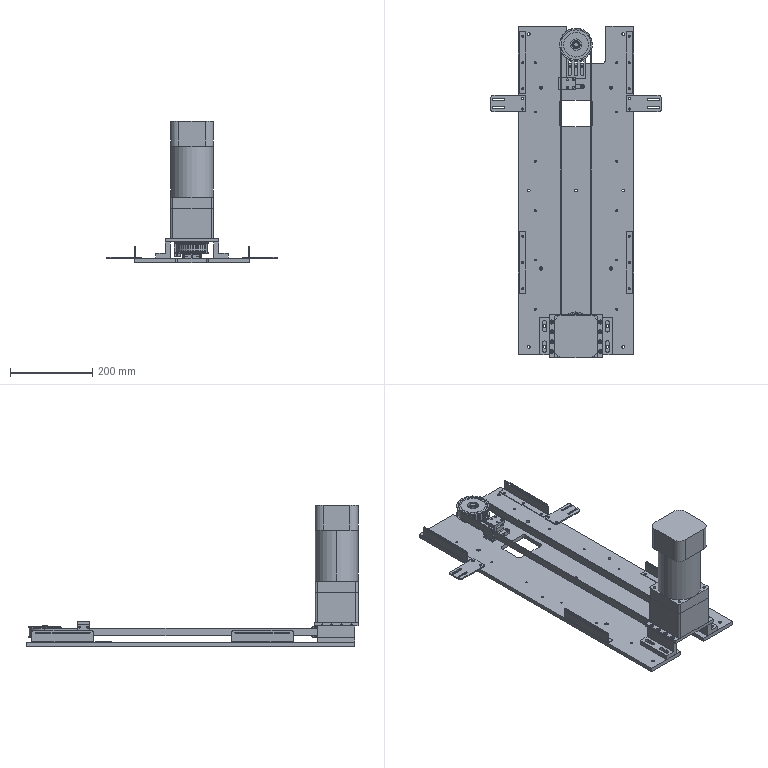Assembly | SolidWorks | mm | 20 component files | 21 solids | 990 faces | box 414 x 807.5 x 343 mm | volume 5377304 mm3 | cylinder 626 | plane 299 | cone 65 | commonest cylinder face diameters 2.94 x86 2.08 x84 5 x54 4.2 x50 10 x46 66.21 x40 71.39 x38 3.3 x36
Bill of materials:
200WBrakeMotor, | 1 |  | Vertical stacked body: square block base, a cylindrical middle section, and a square cap with rounded corners on top; a small round shaft with a short collar sticks out of the base end. The overall form looks like a motor or gearmotor housing.
ATPA18H075 | 1 |  | Toothed pulley-like wheel with flanges at both ends. The toothed cylindrical hub has many axial grooves, there is a central through bore with a counterbore or step on one face, and one radial hole goes through the toothed rim.
'-2 | 1 |  | Toothed pulley-like wheel with end flanges, similar in form to unnamed part, but with a plain bore that has a single rectangular keyway, and with radial holes through the toothed rim.
3 | 1 |  | Short solid cylinder with chamfered ends. One end has a hexagonal socket recess and the other end has a flat circular face inside a chamfer. The form looks like a set screw / grub screw.
DC-024-05 | 2 |  | L-section block: a long, tall upright wall joined to a lower base flange running its full length. The top of the wall has a row of four small holes, and the base flange has two elongated slots.
DC-024-06 | 1 |  | Flat rectangular plate with one large round through hole set toward one end. Four larger holes sit near the corners and eight smaller holes run along the two long edges.
DC-024-24 | 1 |  | Rectangular block with three parallel slots at one end and a round bore at the other. A narrow saw cut runs from the bore to the end face, and a cross hole runs through the side, which looks like a split-clamp feature. There is a step on the underside.
DC-024-25 | 1 |  | Stepped cylindrical pin: a larger-diameter base section and a longer, smaller-diameter shank. A narrow circumferential groove sits near the free end of the shank, and the edges are chamfered.
DC-024-29 | 1 |  | Thick L-shaped angle bracket. The horizontal flange has four larger through holes in a rectangular pattern, and the vertical leg has four smaller through holes in a rectangular pattern.
DC-024-30 | 1 |  | Flat rectangular plate with four round through holes, one near each corner.
DC-024-31 | 4 |  | Long, thin angle bracket (L-section). The tall vertical leg has a long slot with rounded ends running nearly its full length and rounded top corners. The short horizontal flange has three round holes along its length.
DC-024-39 | 1 |  | Rectangular bar with chamfered vertical corners, which gives an elongated octagonal outline in plan. Two vertical through holes near the ends appear counterbored, and one horizontal cross hole goes through the long side at the middle.
DC-024-40 | 1 |  | Long, thin, flat rectangular plate. Each short end has a rectangular notch with rounded corners, so the plate's outline looks roughly like an H or a double U. There is one rounded-rectangle through-cutout near one end, and many small round through-holes are spread over the face.
DC-024-43 | 2 |  | Flat rectangular plate with rounded corners. Two round through-holes sit near one short edge, and two parallel elongated slots with rounded ends run lengthwise near the opposite short edge.
tongbudai | 1 |  | Closed, thin-walled band shaped like an obround (stadium): two straight parallel sides joined by semicircular ends. It is open at the top and bottom, with no floor or cover.
Mates:
1. coincident | DC-024-05-1 face at (-90.633, -439.091, 53) dir (0, 0, 1) | DC-024-06-1 face at (-25.633, -394.091, 53) dir (0, 0, -1)
2. coincident | DC-024-05-1 face at (-90.633, -439.091, 25) dir (-1, 0, 0) | DC-024-06-1 face at (-90.633, -446.591, 61) dir (-1, 0, 0)
3. width | 200WBrakeMotor,-1 face at (26.367, -342.591, 134) dir (1, 0, 0) | 200WBrakeMotor,-1 face at (-77.633, -342.591, 134) dir (-1, 0, 0) | DC-024-05-1 face at (-90.633, -439.091, 25) dir (-1, 0, 0) | DC-024-05-2 face at (39.367, -349.091, 25) dir (1, 0, 0)
4. coincident | DC-024-06-1 face at (39.367, -446.591, 61) dir (0, -1, 0) | 200WBrakeMotor,-1 face at (-77.633, -446.591, 134) dir (0, -1, 0)
5. coincident | DC-024-06-1 face at (-25.633, -394.091, 61) dir (0, 0, 1) | 200WBrakeMotor,-1 face at (-25.633, -394.591, 61) dir (0, 0, -1)
6. coincident | ATPA18H075-A-N20-1/-2-1 face at (-22.284, -394.309, 51.5) dir (0, 0, 1) | ATPA18H075-1 face at (-43.362, 325.7, 51.5) dir (0, 0, 1)
7. concentric | DC-024-24-1 face at (-25.633, 315.409, -17.713) dir (0, 0, 1) r 7.5 | ATPA18H075-1 face at (-25.633, 315.409, 5.216) dir (0, 0, 1) r 10
8. concentric | DC-024-24-1 face at (-25.633, 315.409, -17.713) dir (0, 0, 1) r 7.5 | DC-024-25-1 face at (-25.633, 315.409, 54.5) dir (0, 0, -1) r 6
9. coincident | tongbudai-1 face at (-61.333, 315.409, 48) dir (1, 0, 0) | DC-024-29-1 face at (-61.333, 205.806, 63) dir (-1, 0, 0)
10. coincident | DC-024-29-1 face at (-61.333, 235.806, 63) dir (0, 1, 0) | DC-024-30-1 face at (-63.333, 235.806, 18) dir (0, 1, 0)
11. coincident | tongbudai-1 face at (-63.333, 315.409, 48) dir (-1, 0, 0) | DC-024-30-1 face at (-63.333, 220.806, 37) dir (1, 0, 0)
12. coincident | DC-024-29-1 face at (-53.333, 205.806, 18) dir (0, 0, -1) | DC-024-30-1 face at (-63.333, 205.806, 18) dir (0, 0, -1)
13. coincident | DC-024-31-1 face at (114.367, 196.909, 42.5) dir (1, 0, 0) | DC-024-31-2 face at (114.367, -289.091, 42.5) dir (1, 0, 0)
14. coincident | DC-024-31-1 face at (112.867, 196.909, 13) dir (0, 0, -1) | DC-024-31-2 face at (112.867, -289.091, 13) dir (0, 0, -1)
15. coincident | DC-024-05-2 face at (39.367, -349.091, 25) dir (1, 0, 0) | DC-024-06-1 face at (39.367, -446.591, 61) dir (1, 0, 0)
16. width | DC-024-05-2 face at (27.367, -439.091, 13) dir (0, -1, 0) | DC-024-05-2 face at (27.367, -349.091, 13) dir (0, 1, 0) | DC-024-06-1 face at (39.367, -341.591, 61) dir (0, 1, 0) | DC-024-06-1 face at (39.367, -446.591, 61) dir (0, -1, 0)
17. coincident | DC-024-05-2 face at (39.367, -349.091, 53) dir (0, 0, 1) | DC-024-06-1 face at (-25.633, -394.091, 53) dir (0, 0, -1)
18. coincident | DC-024-05-1 face at (-113.633, -439.091, 13) dir (0, 0, -1) | DC-024-40-1 face at (-25.633, -9.091, 13) dir (0, 0, 1)
19. coincident | DC-024-05-1 face at (-78.633, -439.091, 13) dir (0, -1, 0) | DC-024-40-1 face at (114.367, -439.091, 13) dir (0, -1, 0)
20. width | DC-024-05-2 face at (39.367, -349.091, 25) dir (1, 0, 0) | DC-024-05-1 face at (-90.633, -439.091, 25) dir (-1, 0, 0) | DC-024-40-1 face at (-165.633, -439.091, 13) dir (-1, 0, 0) | DC-024-40-1 face at (114.367, -439.091, 13) dir (1, 0, 0)
21. coincident | DC-024-31-1 face at (112.867, 196.909, 13) dir (0, 0, -1) | DC-024-40-1 face at (-25.633, -9.091, 13) dir (0, 0, 1)
22. coincident | DC-024-31-1 face at (114.367, 196.909, 42.5) dir (1, 0, 0) | DC-024-40-1 face at (114.367, -439.091, 13) dir (1, 0, 0)
23. width | DC-024-24-1 face at (-3.133, 233.409, 23.5) dir (1, 0, 0) | DC-024-24-1 face at (-48.133, 233.409, 23.5) dir (-1, 0, 0) | DC-024-40-1 face at (-165.633, -439.091, 13) dir (-1, 0, 0) | DC-024-40-1 face at (114.367, -439.091, 13) dir (1, 0, 0)
24. coincident | DC-024-24-1 face at (-25.633, 283.409, 3.5) dir (0, 0, -1) | DC-024-25-1 face at (-25.633, 315.409, 3.5) dir (0, 0, -1)
25. concentric | tongbudai-1 face at (-25.633, 315.409, 48) dir (0, 0, -1) r 37.7 | ATPA18H075-1 face at (-25.633, 315.409, 38.5) dir (0, 0, 1) r 35.695
26. width | tongbudai-1 face at (-25.633, 315.409, 48) dir (0, 0, 1) | tongbudai-1 face at (-25.633, 315.409, 29) dir (0, 0, -1) | ATPA18H075-1 face at (-56.802, 333.502, 49) dir (0, 0, -1) | ATPA18H075-1 face at (-56.802, 333.502, 28) dir (0, 0, 1)
27. concentric | ATPA18H075-A-N20-1/-2-1 face at (-25.633, -374.591, 38.5) dir (0, 0, -1) r 35.695 | tongbudai-1 face at (-25.633, -374.591, 48) dir (0, 0, -1) r 37.7
28. coincident | DC-024-40-1 face at (-25.633, -9.091, 13) dir (0, 0, 1) | DC-024-39-1 face at (-25.633, 213.409, 13) dir (0, 0, -1)
29. width | DC-024-39-1 face at (-45.633, 208.409, 23) dir (-1, 0, 0) | DC-024-39-1 face at (-5.633, 208.409, 23) dir (1, 0, 0) | DC-024-24-1 face at (-3.133, 233.409, 23.5) dir (1, 0, 0) | DC-024-24-1 face at (-48.133, 233.409, 23.5) dir (-1, 0, 0)
30. distance | DC-024-39-1 face at (-5.633, 218.409, 23) dir (0, 1, 0) | DC-024-24-1 face at (-3.133, 233.409, 23.5) dir (0, -1, 0)
31. coincident | DC-024-05-1 face at (-78.633, -439.091, 13) dir (0, -1, 0) | DC-024-05-2 face at (27.367, -439.091, 13) dir (0, -1, 0)
32. distance | DC-024-31-2 face at (112.867, -289.091, 14.5) dir (0, -1, 0) | DC-024-40-1 face at (114.367, -439.091, 13) dir (0, -1, 0)
33. coincident | DC-024-40-1 face at (-25.633, -9.091, 13) dir (0, 0, 1) | DC-024-43-1 face at (138.867, 171.909, 13) dir (0, 0, -1)
34. distance | DC-024-43-1 face at (96.367, 151.909, 16) dir (-1, 0, 0) | DC-024-40-1 face at (114.367, -439.091, 13) dir (1, 0, 0)
35. distance | DC-024-43-1 face at (181.367, 191.909, 16) dir (0, 1, 0) | DC-024-31-1 face at (112.867, 196.909, 14.5) dir (0, -1, 0)